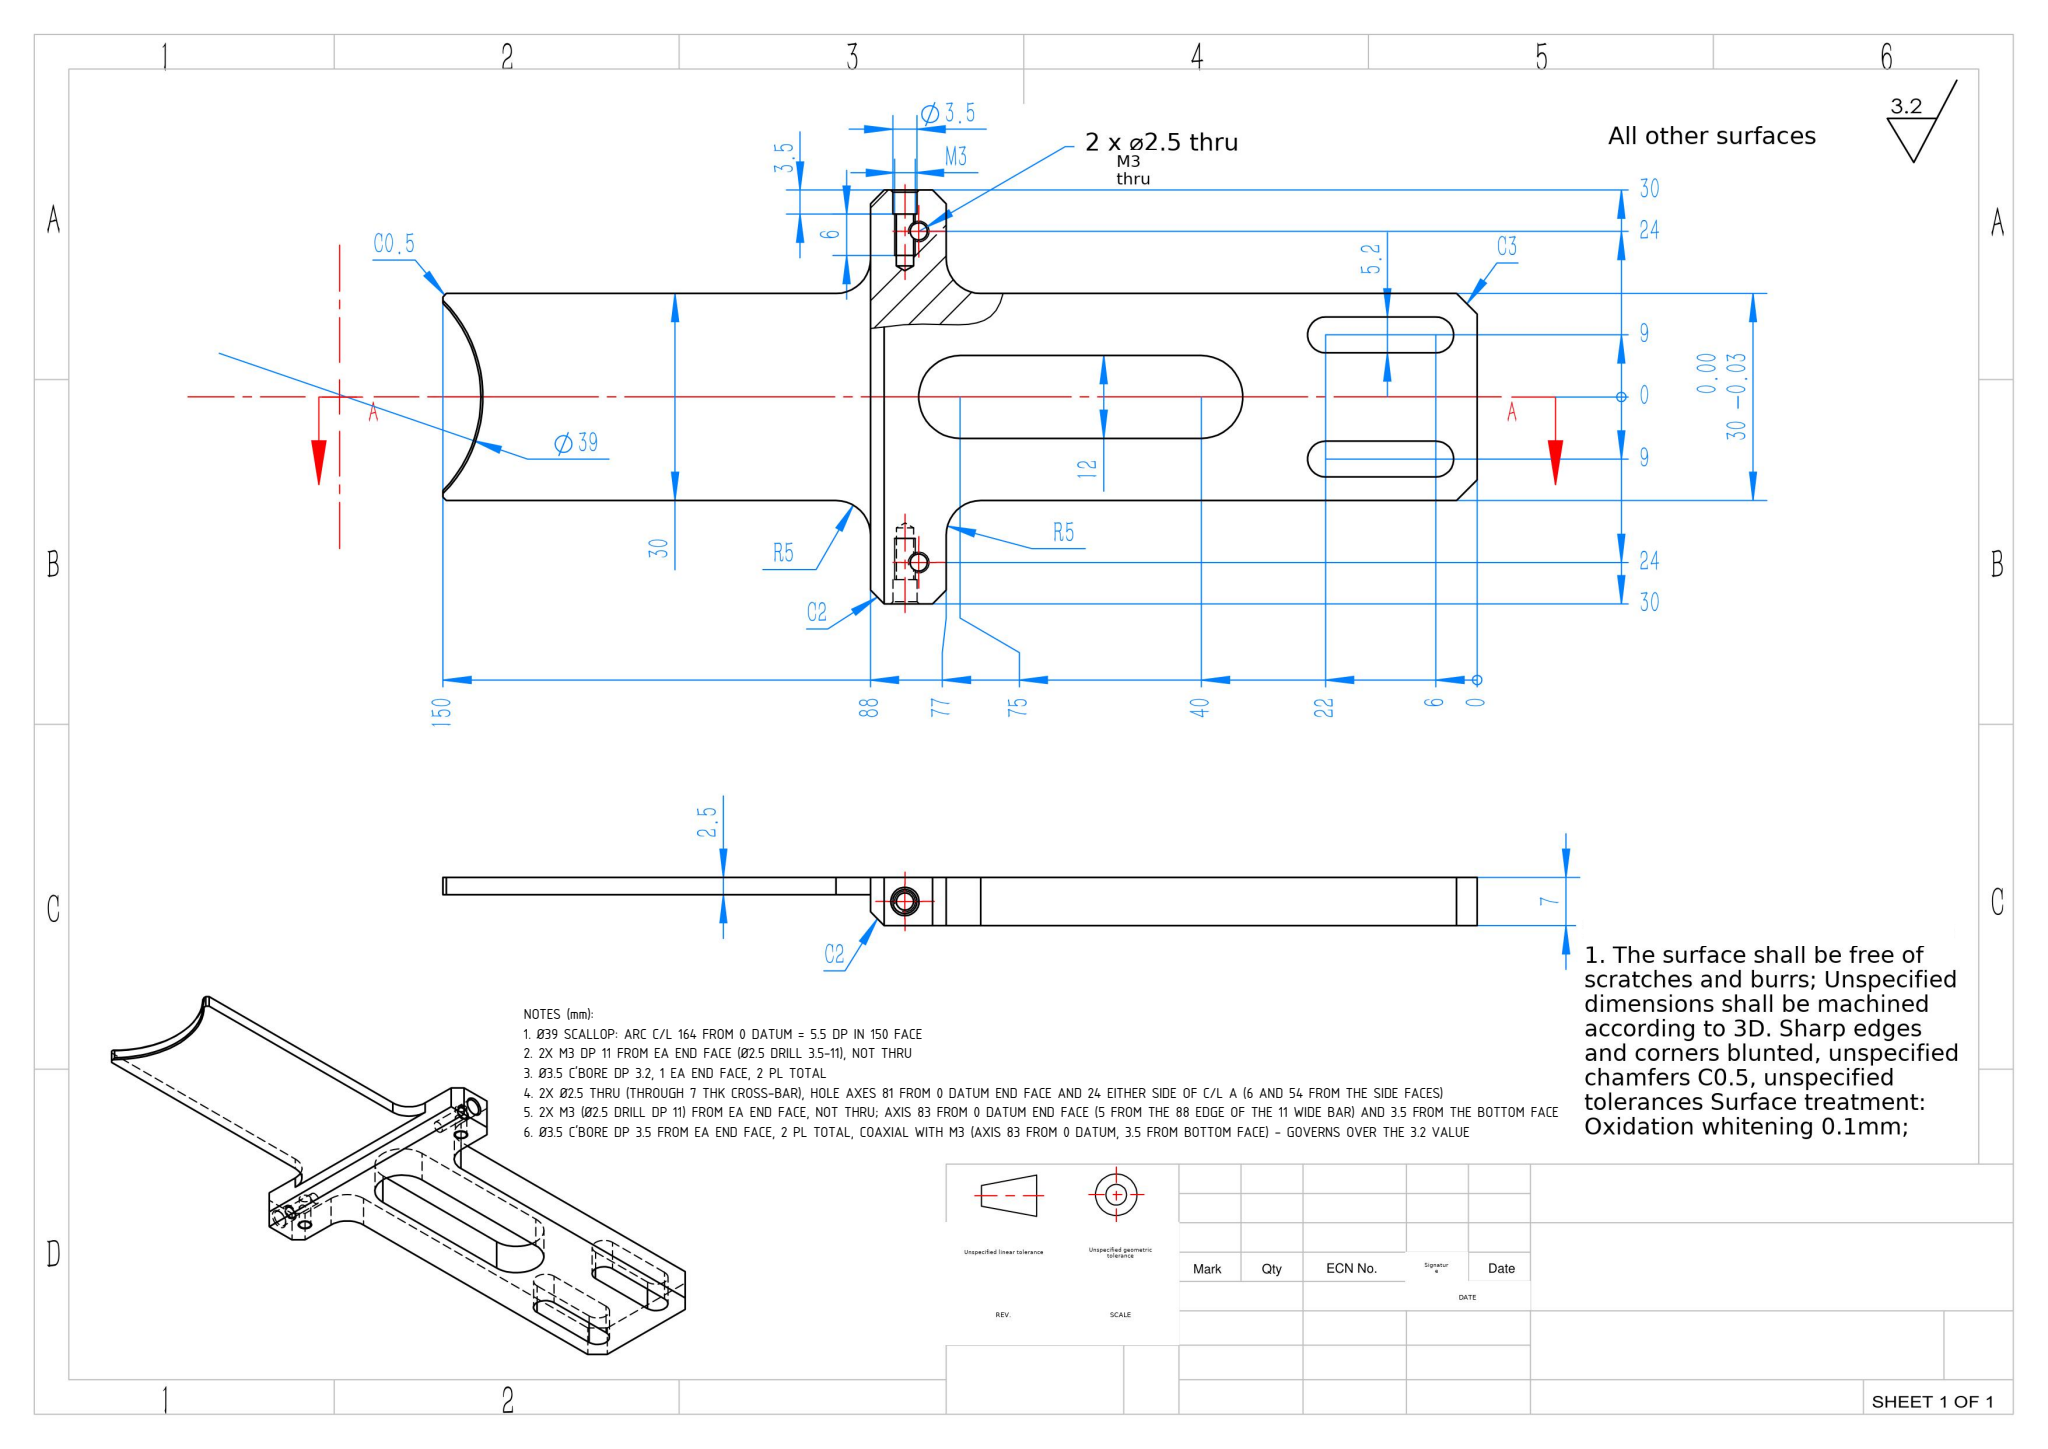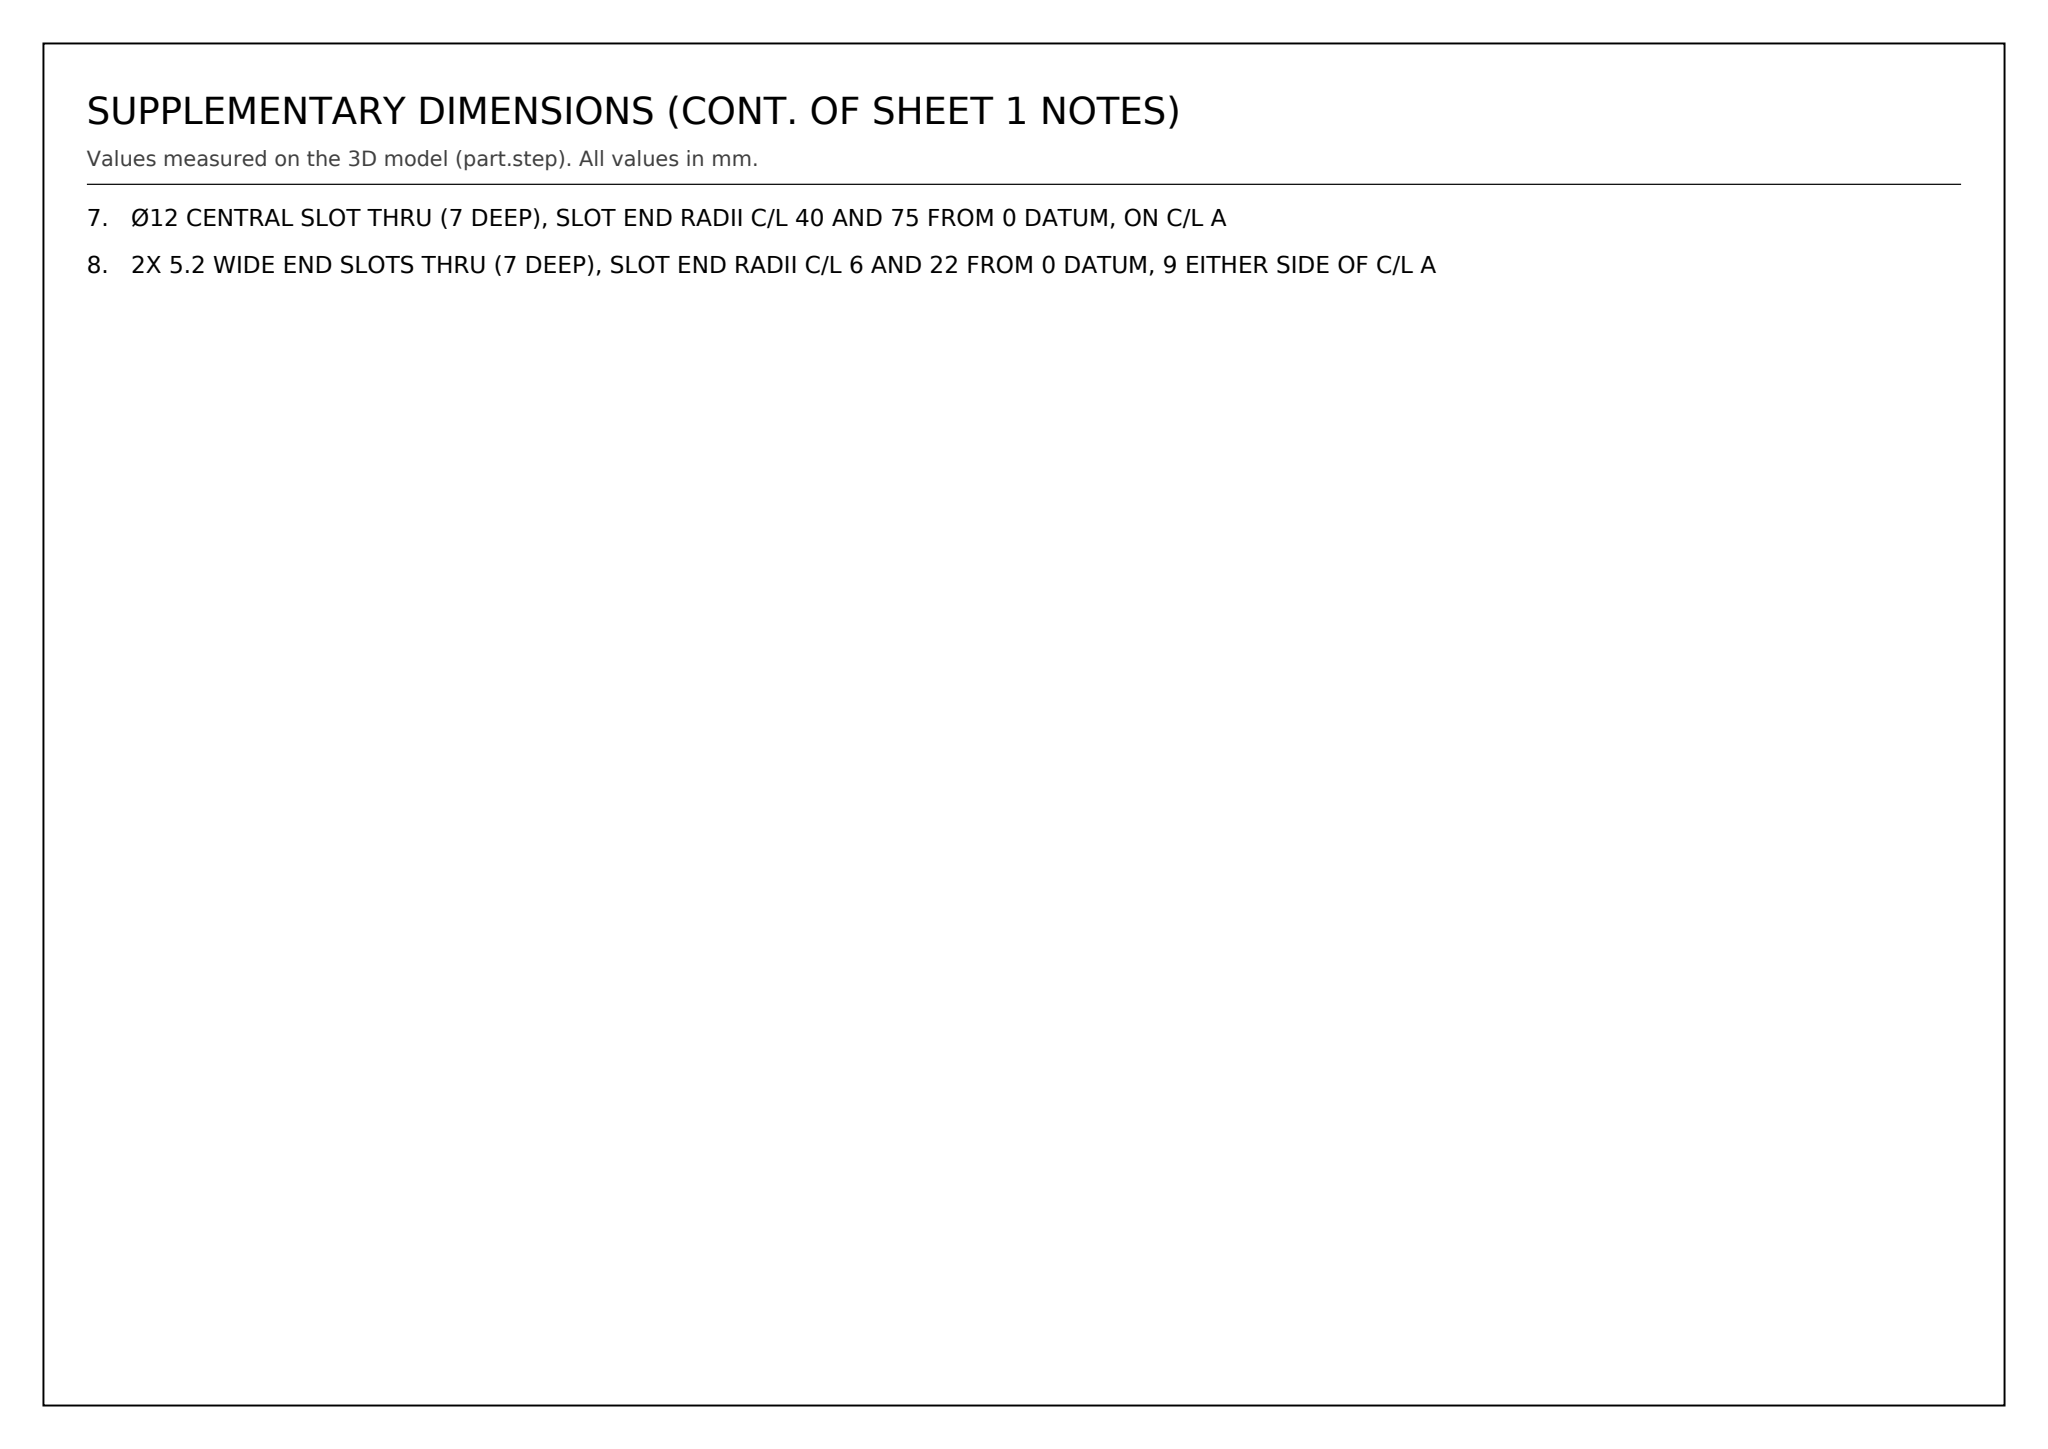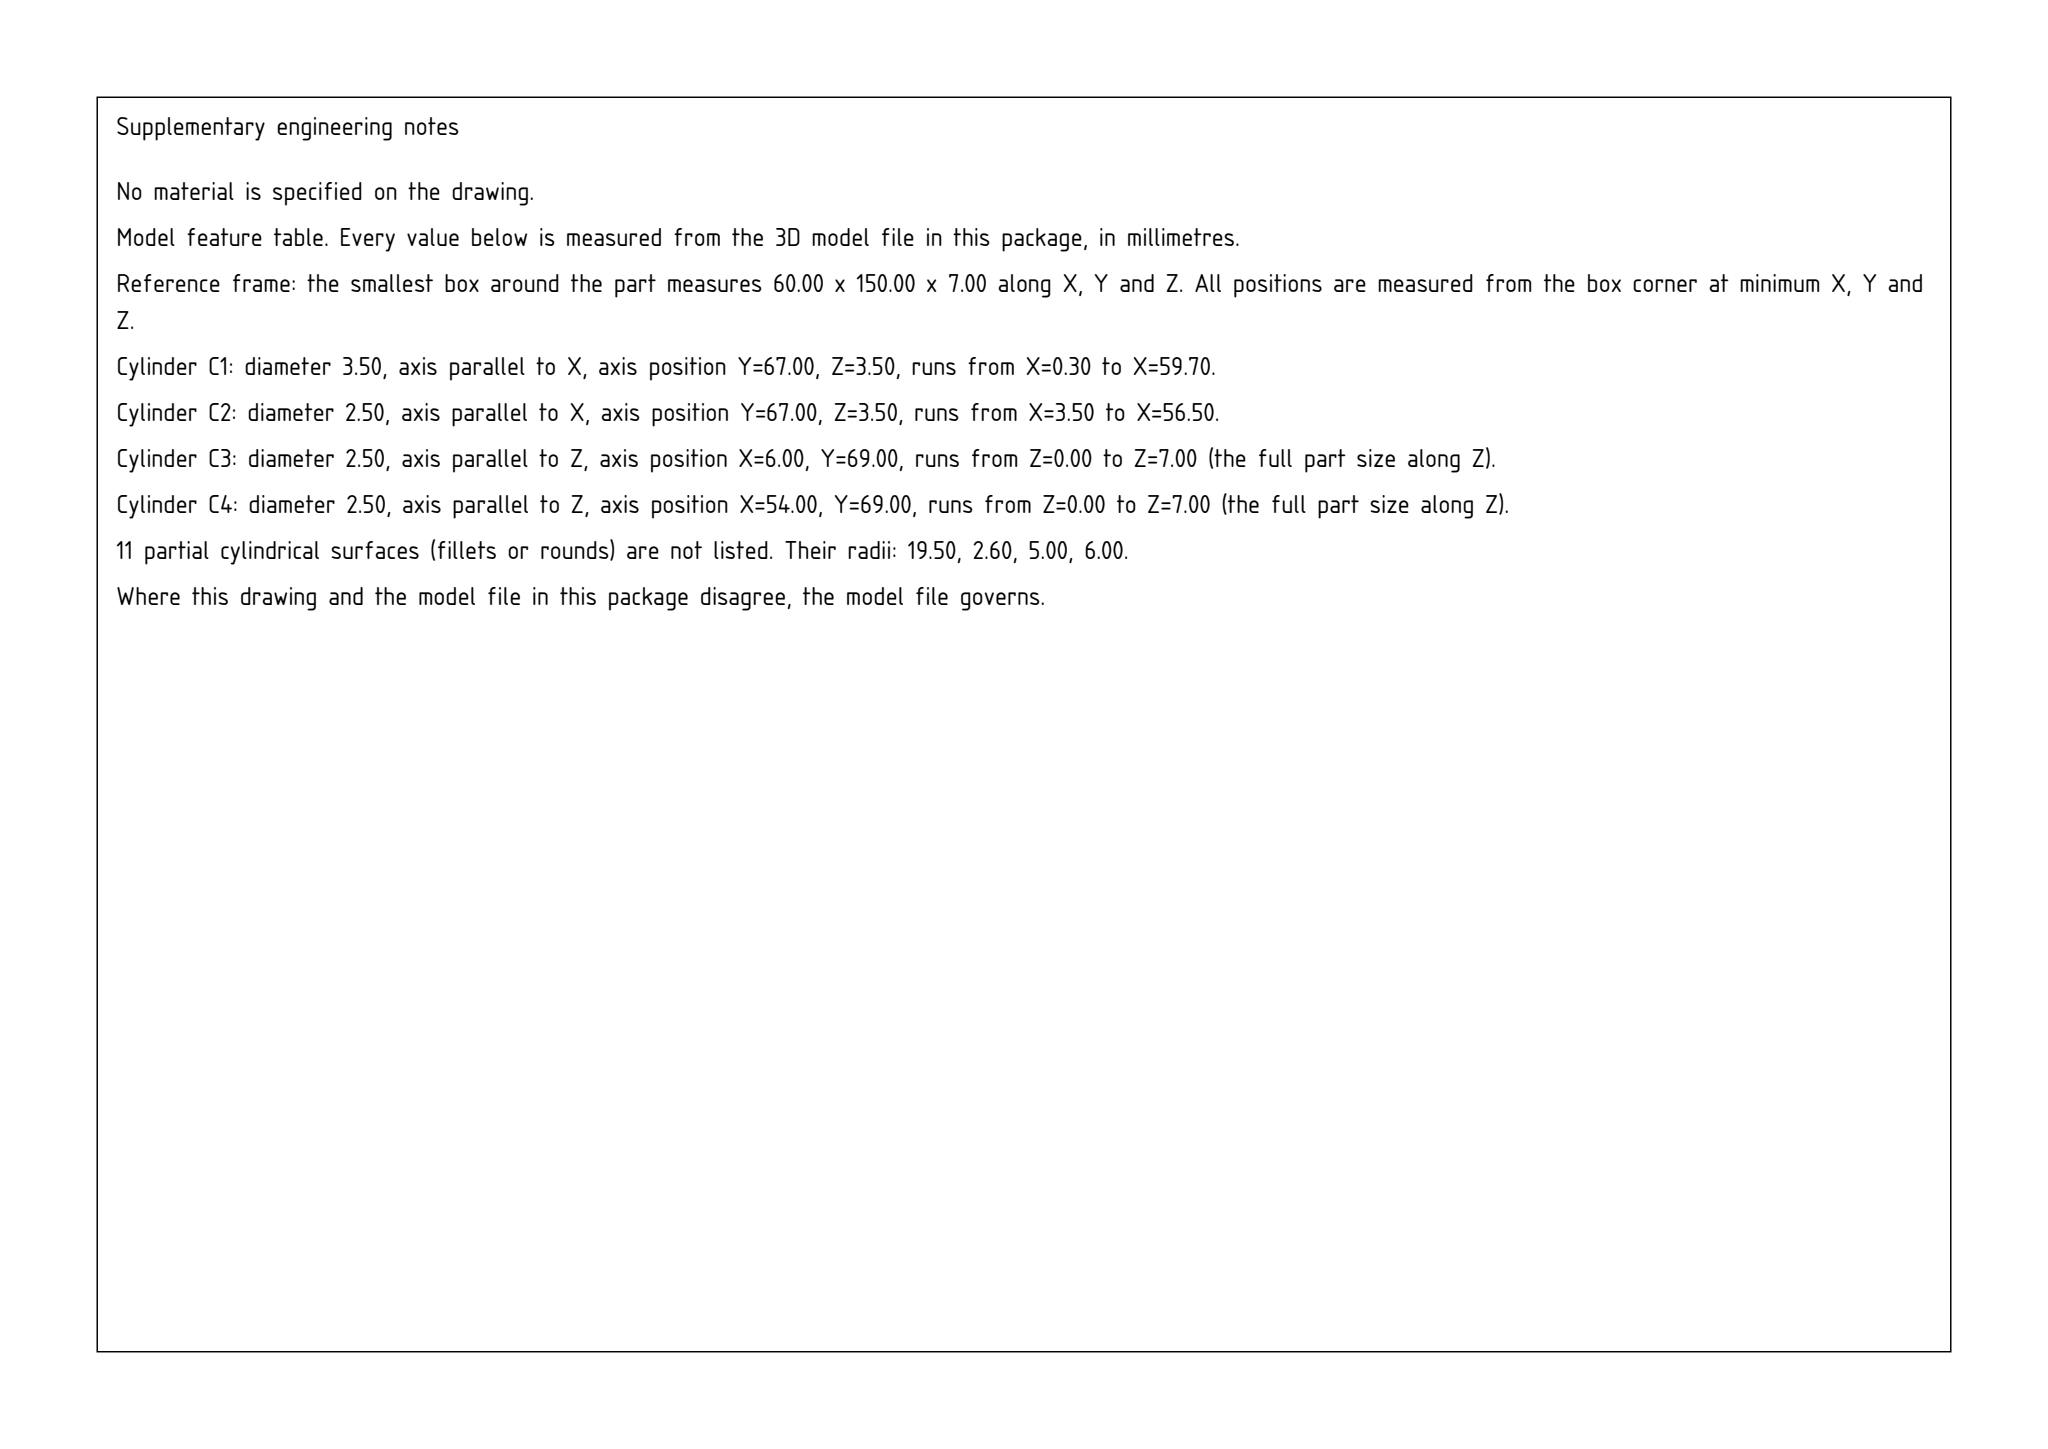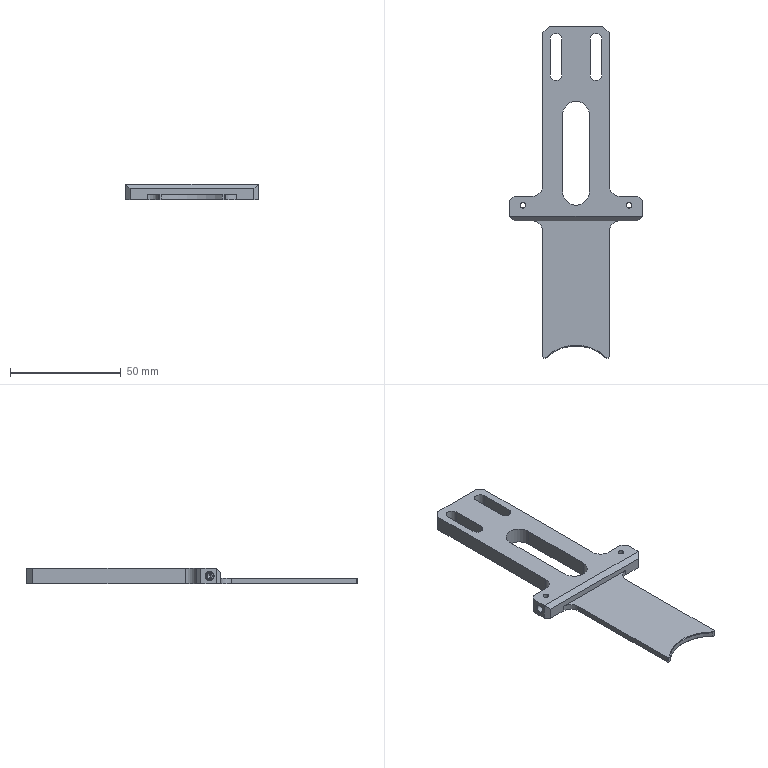Part | SolidWorks | mm | 1 solid | 65 faces | box 60 x 150 x 7 mm | volume 19643 mm3 | plane 32 | cylinder 23 | cone 10 | commonest cylinder face diameters 2.5 x8 3.5 x4 5.2 x4 10 x4 12 x2 39 x1
Drawing notes:
Ø39 SCALLOP: ARC C/L 164 FROM 0 DATUM = 5.5 DP IN 150 FACE | from the solid: Ø39 z-axis cyl at y=-13.79 -> 150.21+13.79=164; 164-19.5=144.5, 150-144.5=5.5
2X M3 DP 11 FROM EA END FACE (Ø2.5 DRILL 3.5-11), NOT THRU | from the solid: cylinders: Ø2.5 x-axis holes at y67.2 z3.5, from x=3.5 to 11.0 and from x=49.0 to 56.5 (bbox x 0-60); not through 60 length
Ø3.5 C'BORE DP 3.2, 1 EA END FACE, 2 PL TOTAL | from the solid: cylinders: Ø3.5 x-axis bores at y67.2 z3.5, x=0.3-3.5 and x=56.5-59.7 (3.2 deep each), only 2 instances
2X Ø2.5 THRU (THROUGH 7 THK CROSS-BAR), HOLE AXES 81 FROM 0 DATUM END FACE AND 24 EITHER SIDE OF C/L A (6 AND 54 FROM THE SIDE FACES) | from the solid: cylinders: hole/bore Ø2.5 axis z at [6, 69.2] and [54, 69.2], from z=0.0 to z=7.0; bbox_xyz 60 x 150.212 x 7 (0 datum end = y 150.2)
2X M3 (Ø2.5 DRILL DP 11) FROM EA END FACE, NOT THRU; AXIS 83 FROM 0 DATUM END FACE (5 FROM THE 88 EDGE OF THE 11 WIDE BAR) AND 3.5 FROM THE BOTTOM FACE | from the solid: cylinders: hole/bore Ø2.5 axis x at [y 67.2, z 3.5], from x=3.5 to 11.0 and from x=49.0 to 56.5; bar faces at y=62.2 and y=73.2
Ø3.5 C'BORE DP 3.5 FROM EA END FACE, 2 PL TOTAL, COAXIAL WITH M3 (AXIS 83 FROM 0 DATUM, 3.5 FROM BOTTOM FACE) - GOVERNS OVER THE 3.2 VALUE | from the solid: cylinders: hole/bore Ø3.5 axis x at [y 67.2, z 3.5], from x=0.3 to 3.5 and from x=56.5 to 59.7
Ø12 CENTRAL SLOT THRU (7 DEEP), SLOT END RADII C/L 40 AND 75 FROM 0 DATUM, ON C/L A | from the solid: cylinders: Ø12 concave arcs axis z at [30, 110.2] and [30, 75.2], from z=0.0 to z=7.0; plane z=7.0 and z=0.0 extents
2X 5.2 WIDE END SLOTS THRU (7 DEEP), SLOT END RADII C/L 6 AND 22 FROM 0 DATUM, 9 EITHER SIDE OF C/L A | from the solid: cylinders: Ø5.2 concave arcs axis z at [21, 128.2], [21, 144.2], [39, 128.2], [39, 144.2], from z=0.0 to z=7.0